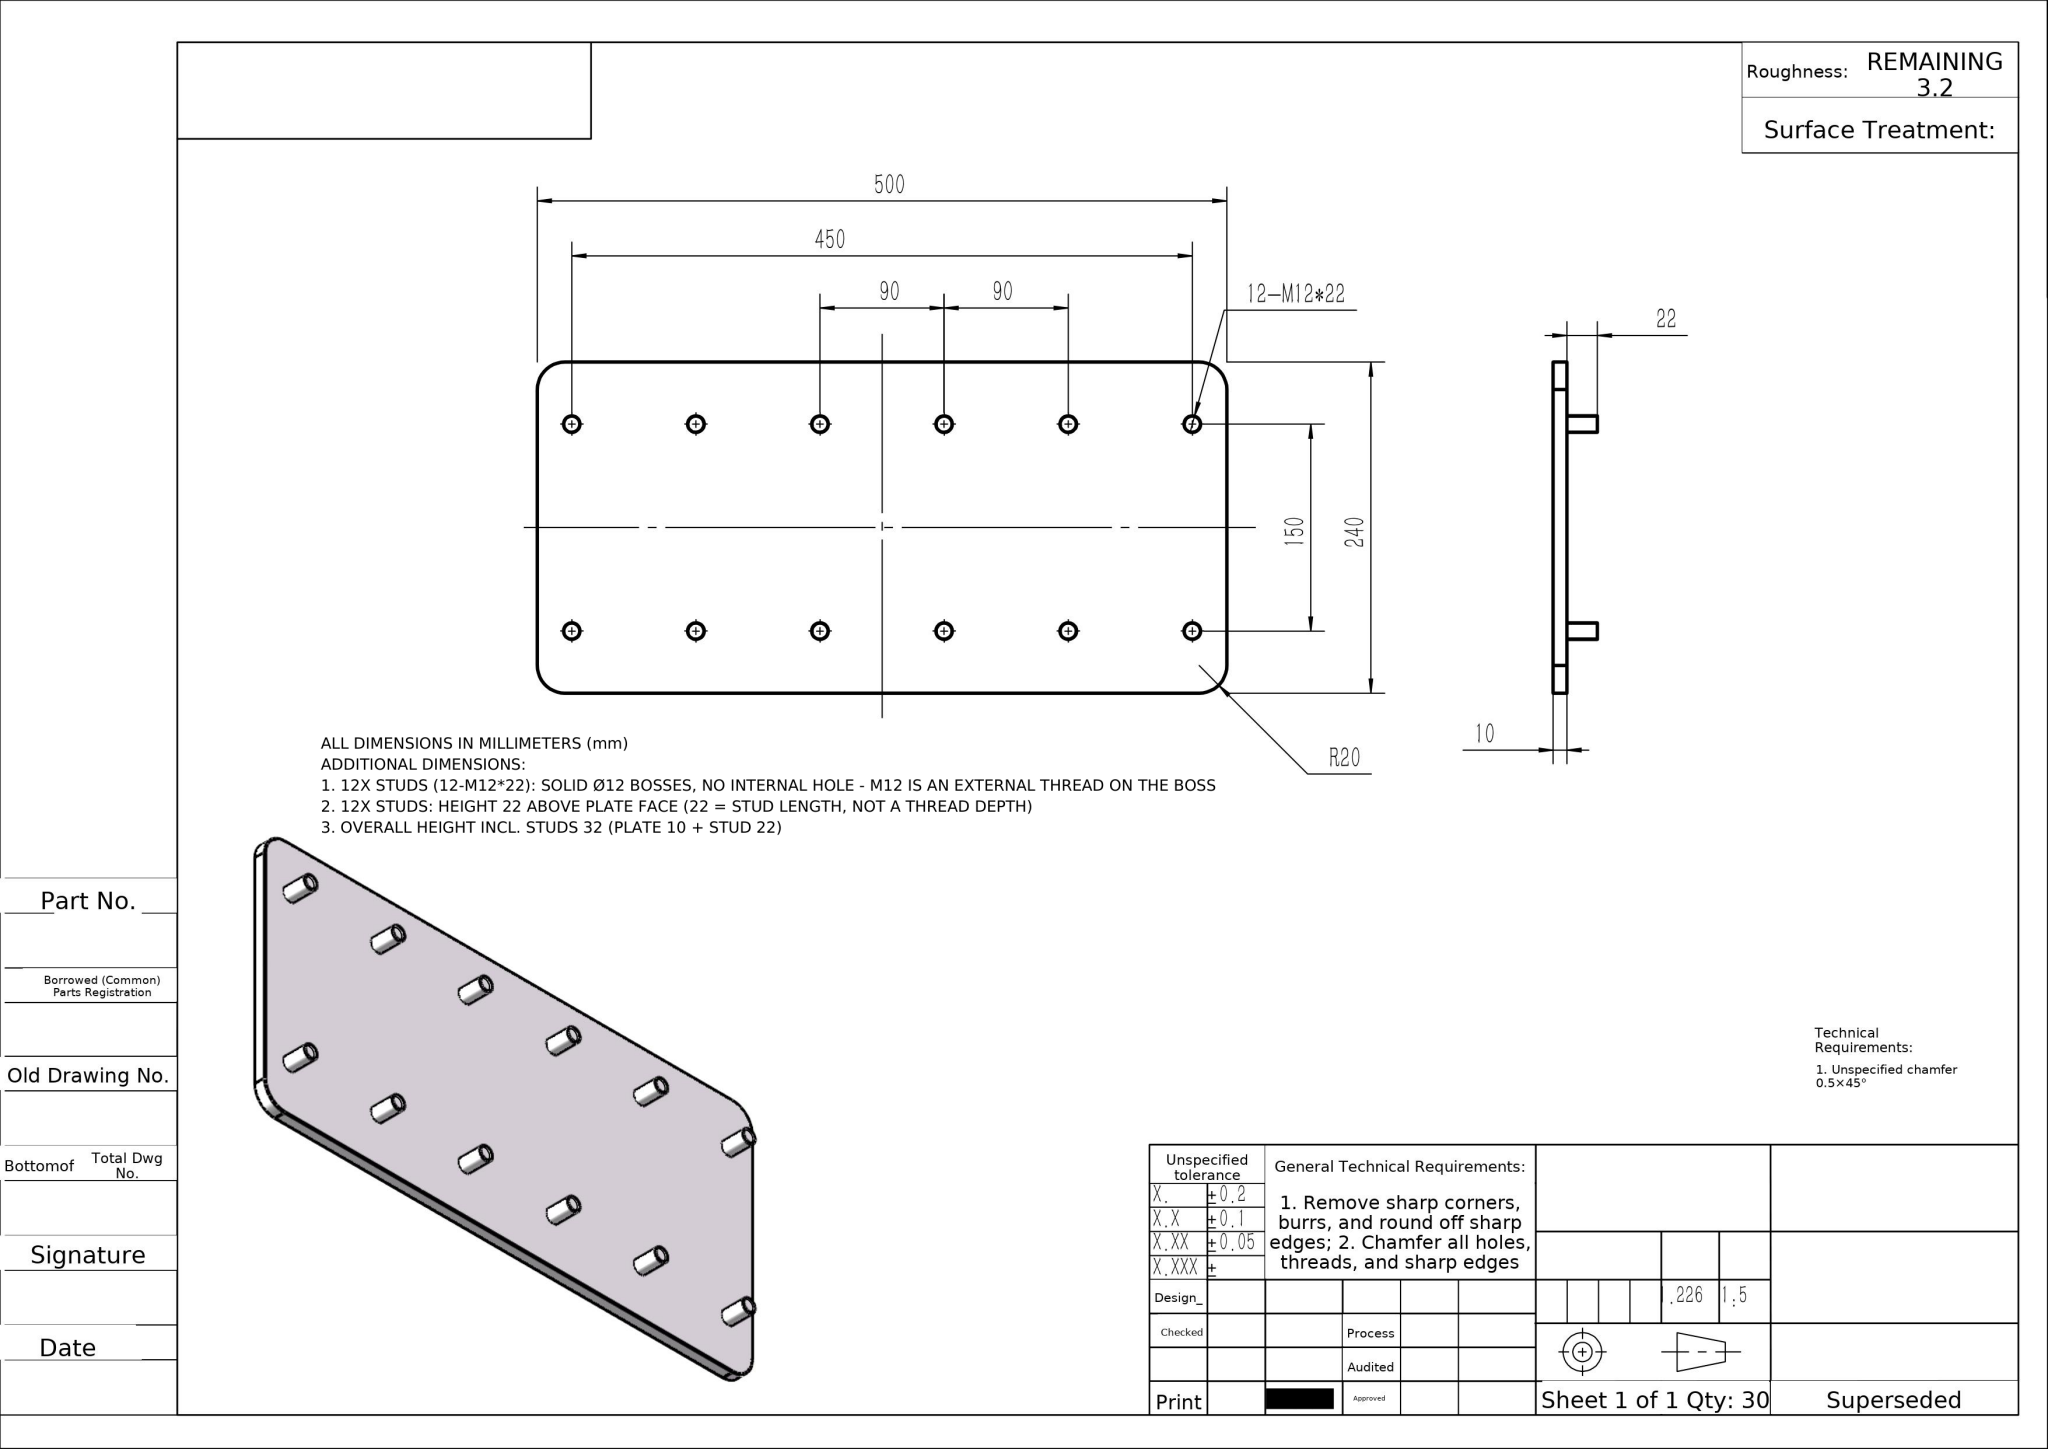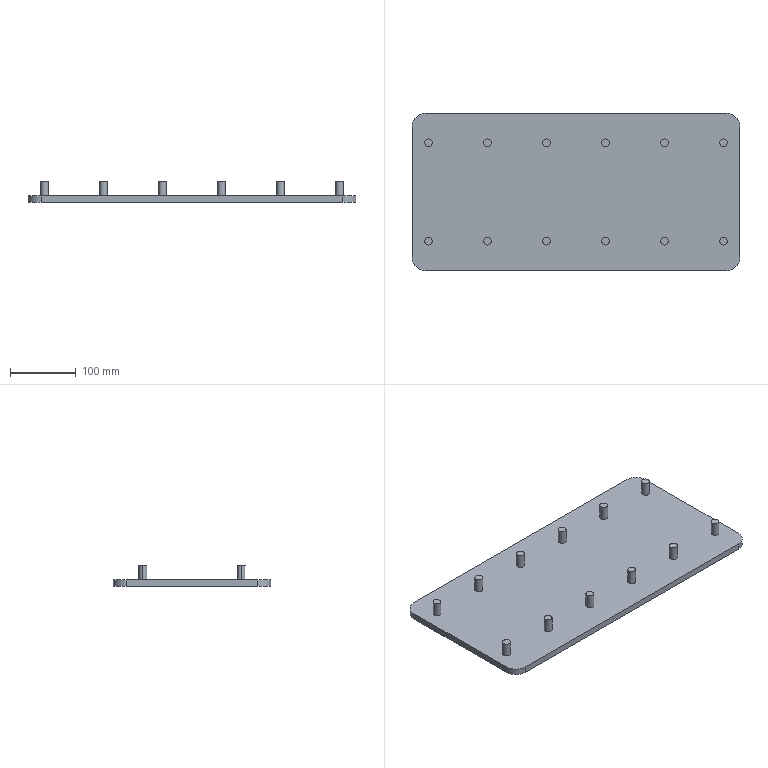Part | NX | mm | 1 solid | 46 faces | box 500 x 240 x 32 mm | volume 1226424 mm3 | cylinder 28 | plane 18 | commonest cylinder face diameters 12 x24 40 x4